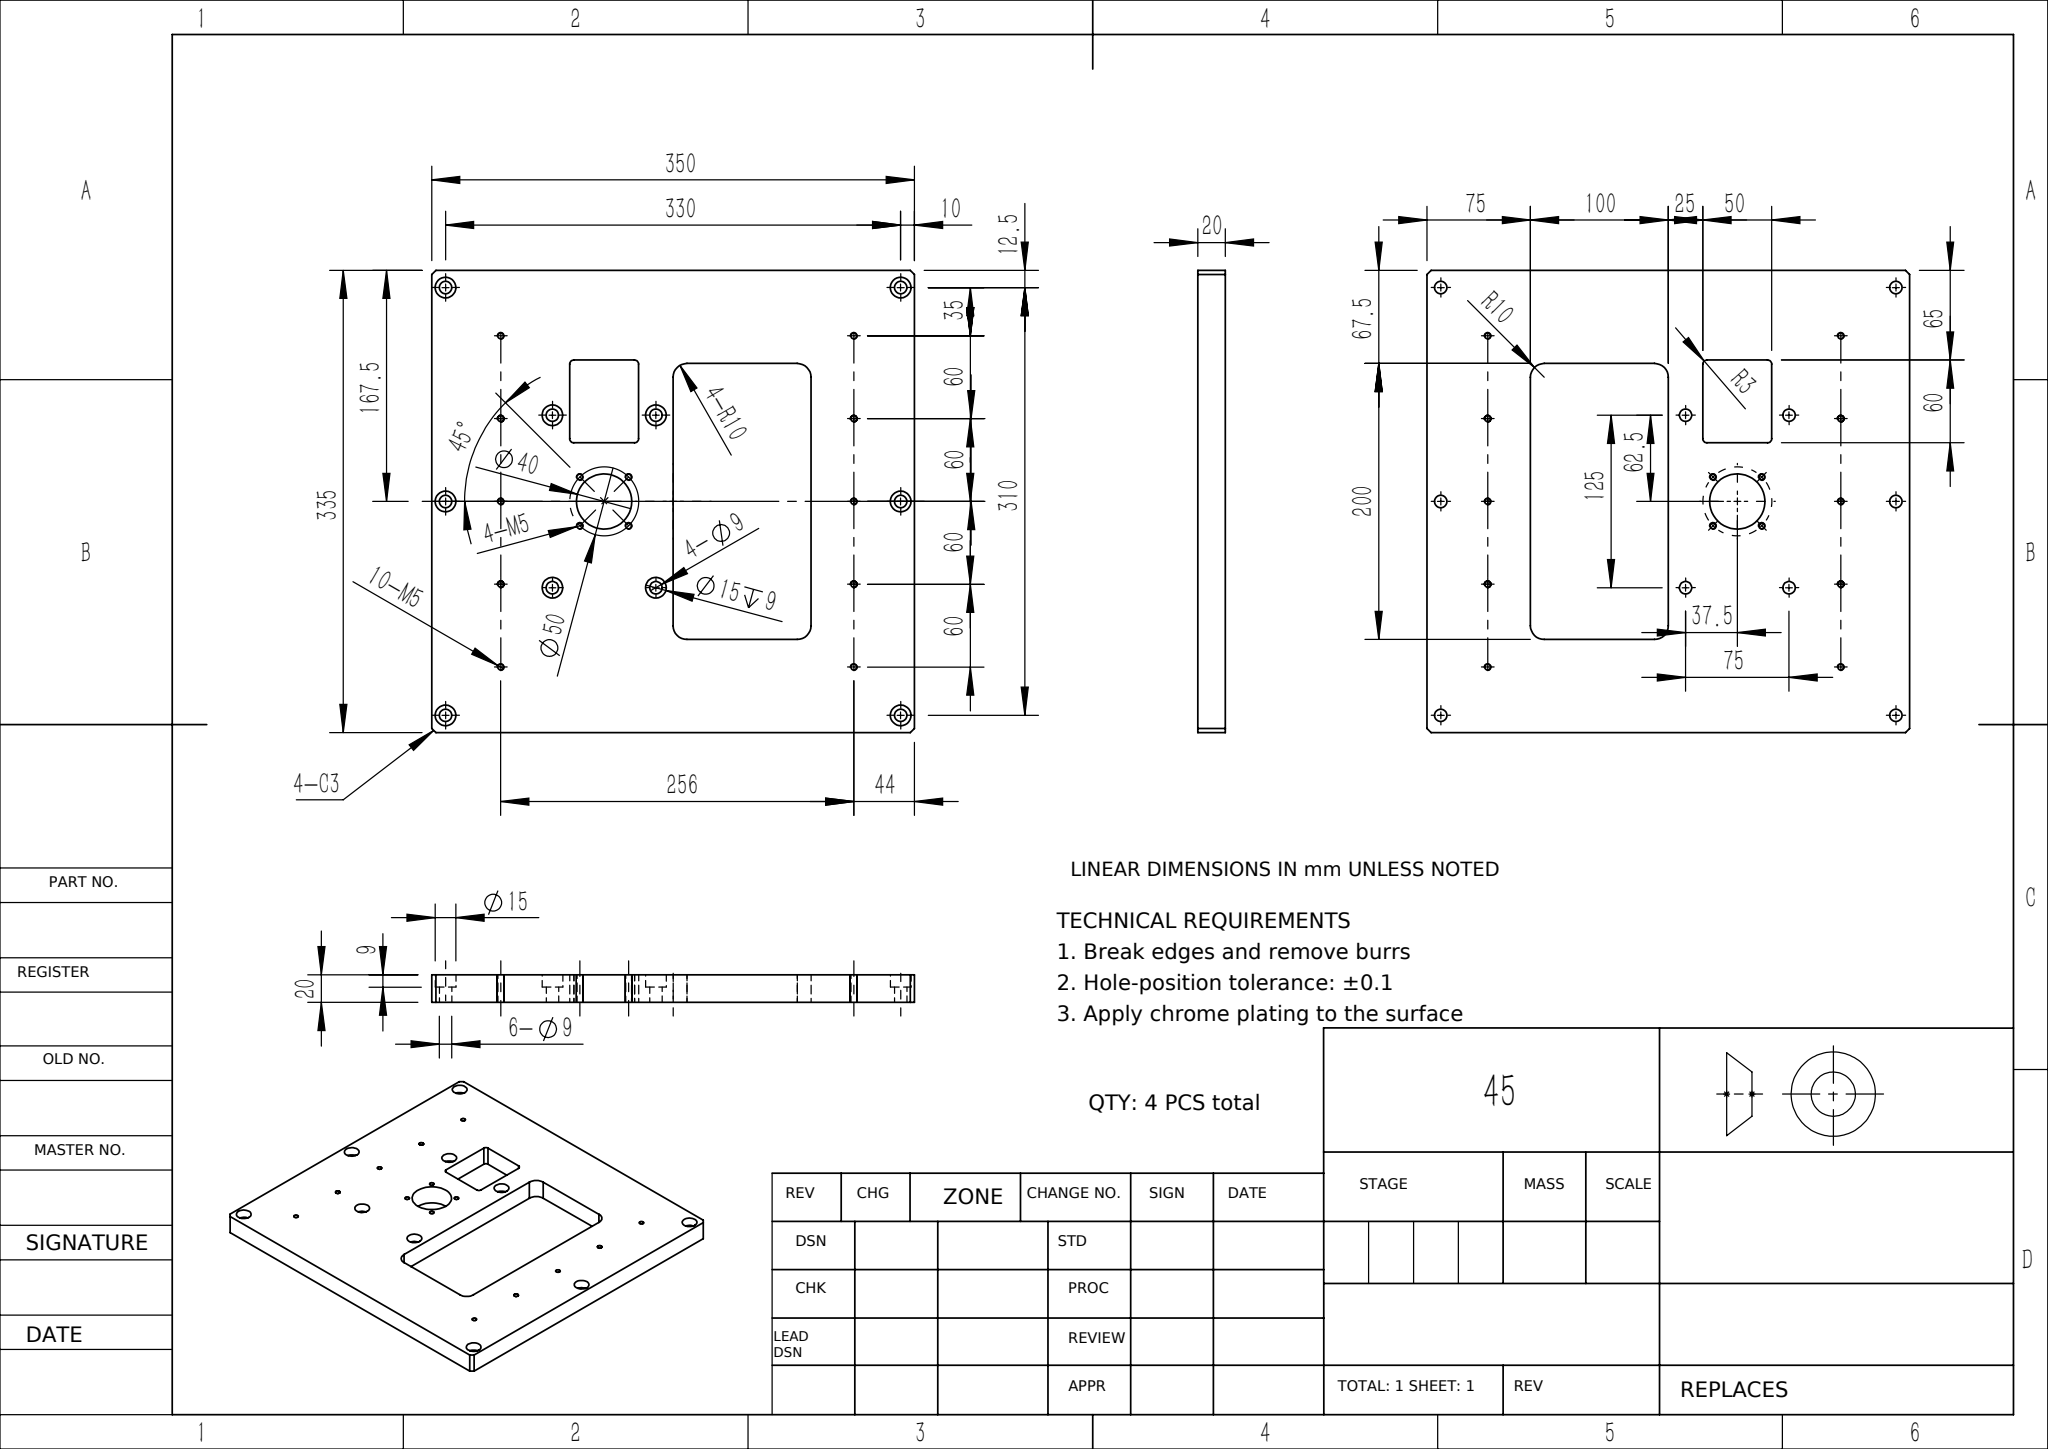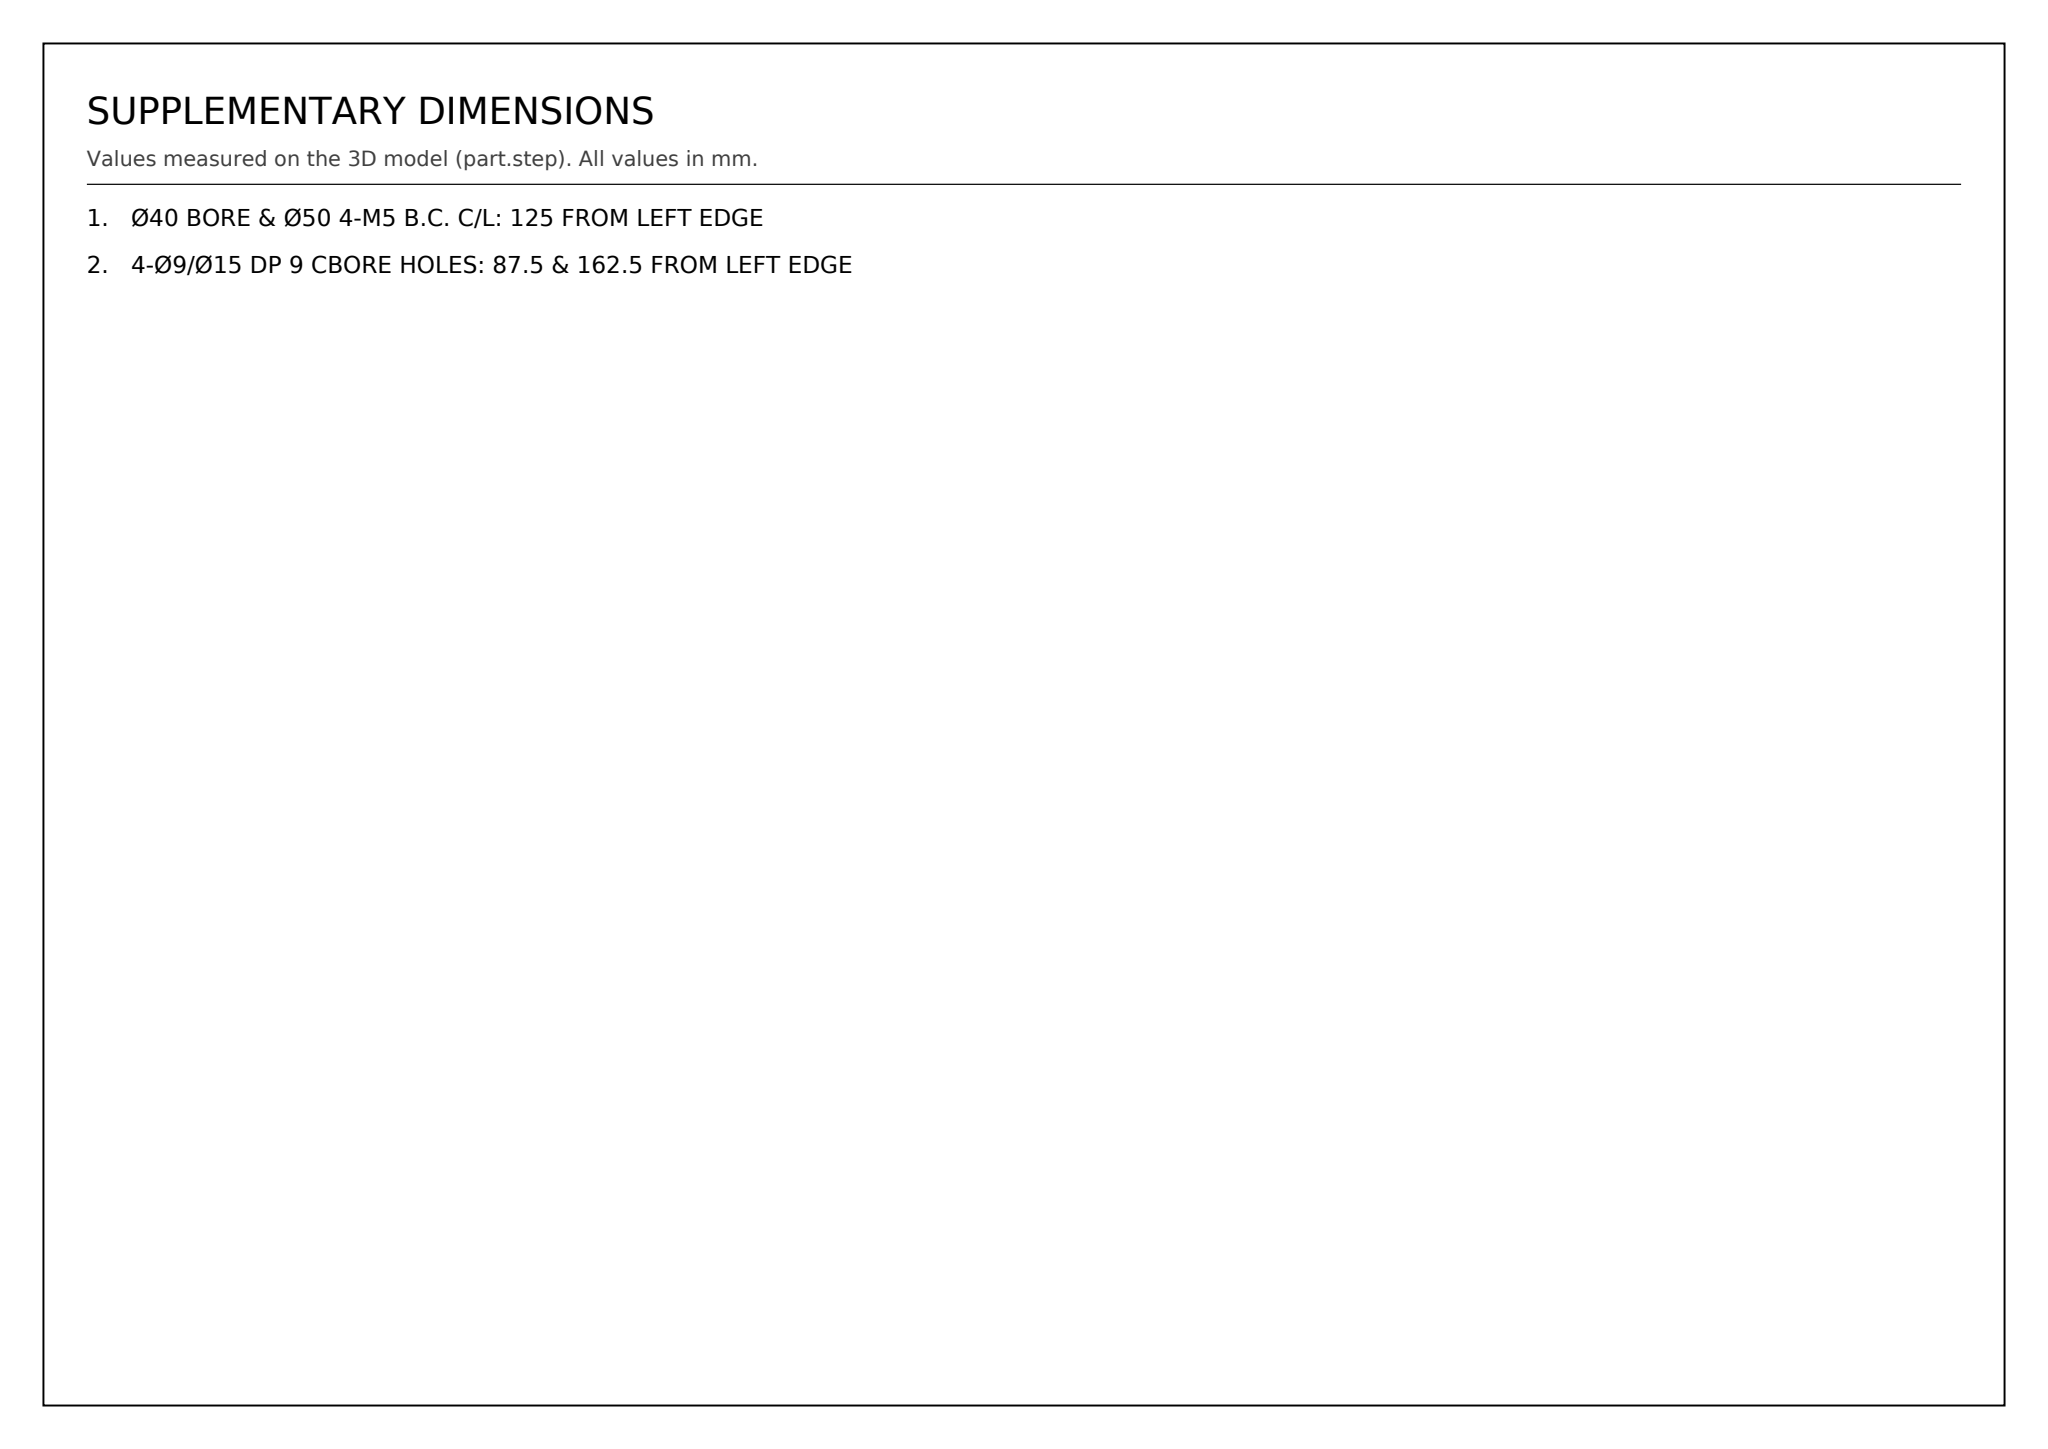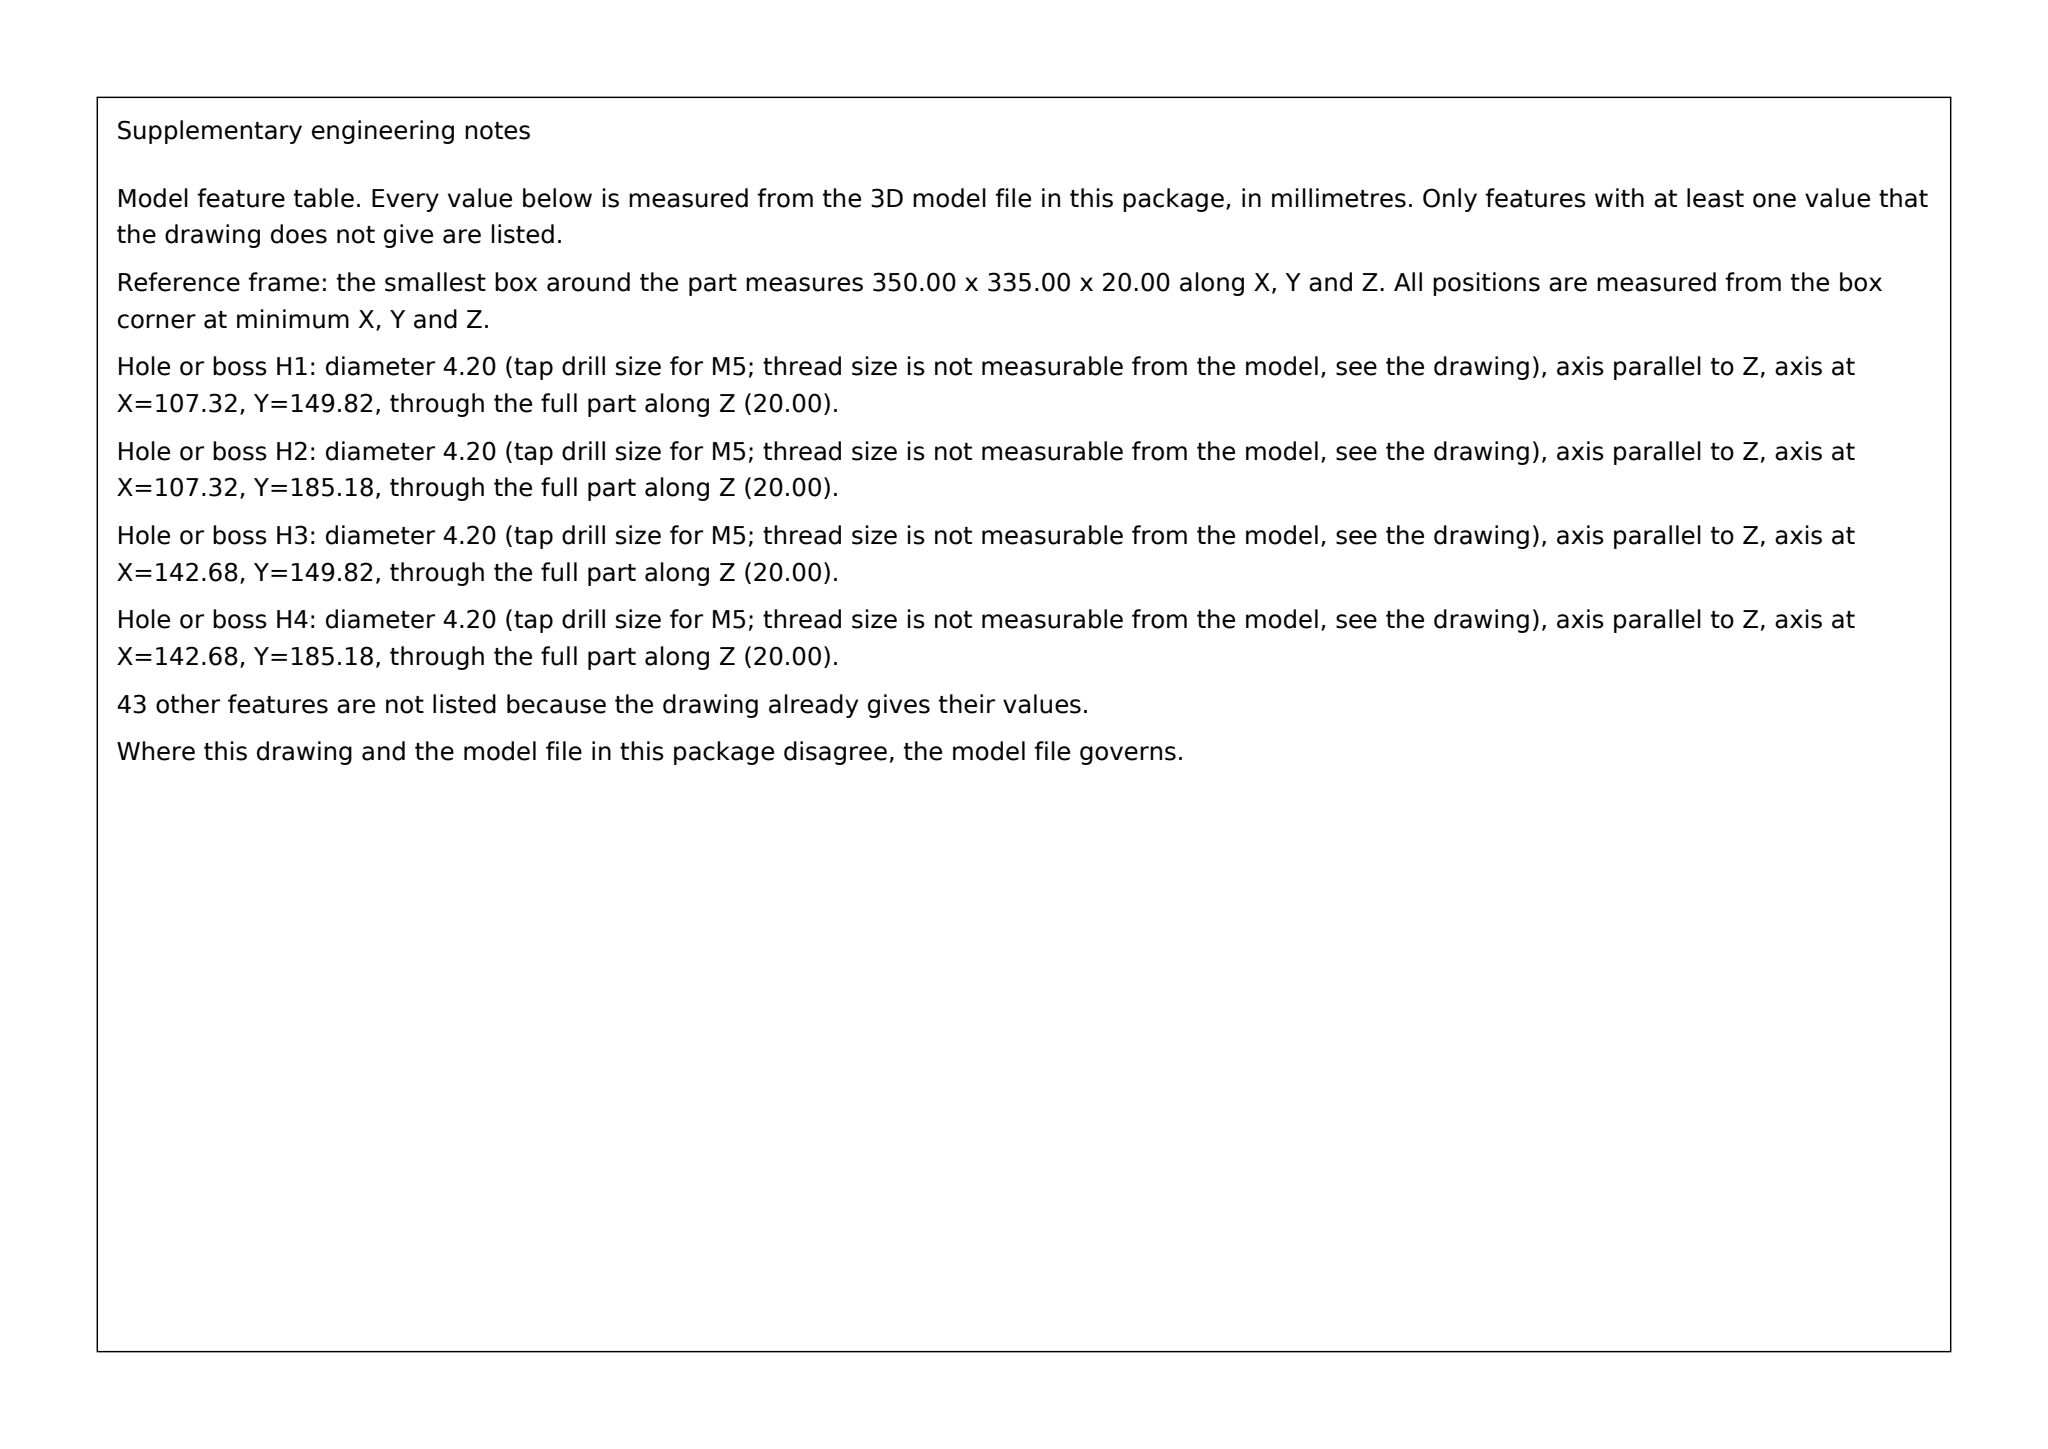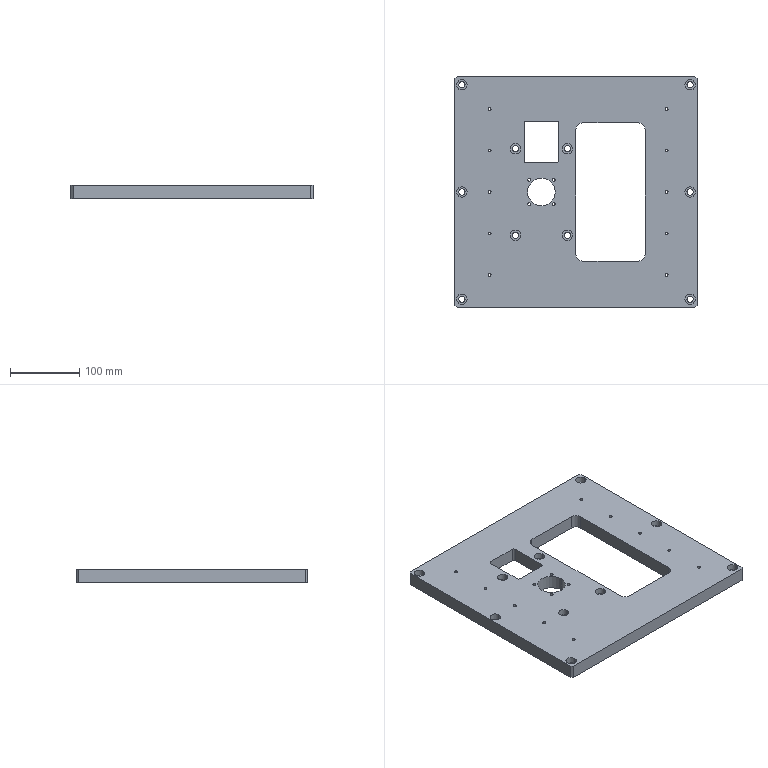Part | SolidWorks | mm | 1 solid | 106 faces | box 350 x 335 x 20 mm | volume 1834597 mm3 | cylinder 78 | plane 28 | commonest cylinder face diameters 4.2 x28 15 x20 9 x20 20 x4 6 x4 40 x2
Drawing notes:
Ø40 BORE & Ø50 4-M5 B.C. C/L: 125 FROM LEFT EDGE | from the solid: Ø40 cyl axis at (125.0, 167.5); M5 Ø4.2 holes at 107.32/142.68 about x=125
4-Ø9/Ø15 DP 9 CBORE HOLES: 87.5 & 162.5 FROM LEFT EDGE | from the solid: Ø9/Ø15 cyls at x=87.5 & 162.5 (y=105 & 230), i.e. 37.5 either side of x=125, 75 apart
build123d program:
from build123d import *

# Parameters (mm, degrees)
SKETCH1_W                                         = 350
SKETCH1_H                                         = 335
BOSS_EXTRUDE1_DEPTH                               = 20
SKETCH2_R                                         = 20
CUT_EXTRUDE1_DEPTH                                = 244.066
M5_TAPPED_HOLE1_D                                 = 4.2
CIRPATTERN1_COUNT                                 = 4
SKETCH5_W                                         = 100
SKETCH5_H                                         = 200
CUT_EXTRUDE2_DEPTH                                = 244.066
FILLET1_R                                         = 10
M5_TAPPED_HOLE2_D                                 = 4.2
LPATTERN1_COUNT                                   = 3
LPATTERN1_PITCH                                   = 60
LPATTERN1_COL_COUNT                               = 3
LPATTERN1_COL_PITCH                               = 60
HOLE_SIZE_ACCORDING_TO_HEX_SOCKET_HEA_D           = 9
HOLE_SIZE_ACCORDING_TO_HEX_SOCKET_HEA_CBORE_D     = 15
HOLE_SIZE_ACCORDING_TO_HEX_SOCKET_HEA_CBORE_DEPTH = 9
CHAMFER1_SIZE                                     = 3
CUT_EXTRUDE3_DEPTH                                = 244.066
HOLE_SIZE_ACCORDING_TO_HEX_SOCKET_2_D             = 9
HOLE_SIZE_ACCORDING_TO_HEX_SOCKET_2_CBORE_D       = 15
HOLE_SIZE_ACCORDING_TO_HEX_SOCKET_2_CBORE_DEPTH   = 9


with BuildPart() as part:
    # Sketch1 → Boss-Extrude1 (new body)
    with BuildSketch(Plane.XY):
        Rectangle(SKETCH1_W, SKETCH1_H)
    extrude(amount=BOSS_EXTRUDE1_DEPTH)

    # Sketch2 → Cut-Extrude1 (cut, through all)
    with BuildSketch(Plane.XY.offset(20)):
        with Locations((-50, 0)):
            Circle(SKETCH2_R)
    extrude(amount=-CUT_EXTRUDE1_DEPTH, mode=Mode.SUBTRACT)

    # M5 Tapped Hole1 (through all)
    with Locations(Plane.XY.offset(20)):
        with Locations((-32.322, 17.678)):
            m5_tapped_hole1 = Hole(M5_TAPPED_HOLE1_D / 2)

    # CirPattern1: M5 Tapped Hole1 ×4 about axis
    cirpattern1_axis = Axis((-50, 0, 0), (0, 0, 1))
    for i in range(1, CIRPATTERN1_COUNT):
        add(m5_tapped_hole1.rotate(cirpattern1_axis, i * 360 / CIRPATTERN1_COUNT), mode=Mode.SUBTRACT)

    # Sketch5 → Cut-Extrude2 (cut, through all)
    with BuildSketch(Plane.XY.offset(20)):
        with Locations((50, 0)):
            Rectangle(SKETCH5_W, SKETCH5_H)
    extrude(amount=-CUT_EXTRUDE2_DEPTH, mode=Mode.SUBTRACT)

    # Fillet1
    fillet1_edges = [part.edges().sort_by_distance(p)[0] for p in [
        (100, 100, 10),
        (100, -100, 10),
        (0, -100, 10),
        (0, 100, 10),
    ]]
    fillet(fillet1_edges, radius=FILLET1_R)

    # M5 Tapped Hole2 (through all)
    with Locations(Plane.XY.offset(20)):
        with Locations((-125, 0), (131, 0)):
            m5_tapped_hole2 = Hole(M5_TAPPED_HOLE2_D / 2)

    # LPattern1: M5 Tapped Hole2 ×3
    with Locations(*[(0, i * LPATTERN1_PITCH, 0) for i in range(1, LPATTERN1_COUNT)]):
        add(m5_tapped_hole2, mode=Mode.SUBTRACT)

    # LPattern1 col: M5 Tapped Hole2 ×3
    with Locations(*[(0, -i * LPATTERN1_COL_PITCH, 0) for i in range(1, LPATTERN1_COL_COUNT)]):
        add(m5_tapped_hole2, mode=Mode.SUBTRACT)

    # Hole Size _ according to_ Hex Socket Hea (through all)
    with Locations(Plane.XY.offset(20)):
        with Locations((165, 155), (-165, 155), (-165, -155), (165, -155), (-165, 0), (165, 0)):
            CounterBoreHole(HOLE_SIZE_ACCORDING_TO_HEX_SOCKET_HEA_D / 2, HOLE_SIZE_ACCORDING_TO_HEX_SOCKET_HEA_CBORE_D / 2, HOLE_SIZE_ACCORDING_TO_HEX_SOCKET_HEA_CBORE_DEPTH)

    # Chamfer1
    chamfer1_edges = [part.edges().sort_by_distance(p)[0] for p in [
        (175, -167.5, 10),
        (-175, -167.5, 10),
        (-175, 167.5, 10),
        (175, 167.5, 10),
    ]]
    chamfer(chamfer1_edges, length=CHAMFER1_SIZE)

    # Sketch10 → Cut-Extrude3 (cut, through all)
    with BuildSketch(Plane.XY.offset(20)):
        with BuildLine():
            Line((-28, 102.5), (-72, 102.5))
            ThreePointArc((-72, 102.5), (-74.121, 101.621), (-75, 99.5))
            Line((-75, 99.5), (-75, 45.5))
            ThreePointArc((-75, 45.5), (-74.121, 43.379), (-72, 42.5))
            Line((-72, 42.5), (-28, 42.5))
            ThreePointArc((-28, 42.5), (-25.879, 43.379), (-25, 45.5))
            Line((-25, 45.5), (-25, 99.5))
            ThreePointArc((-25, 99.5), (-25.879, 101.621), (-28, 102.5))
        make_face()
    extrude(amount=-CUT_EXTRUDE3_DEPTH, mode=Mode.SUBTRACT)

    # Hole Size _ according to_ Hex Socket 2 (through all)
    with Locations(Plane.XY.offset(20)):
        with Locations((-50, 0), (-12.5, -62.5), (-87.5, 62.5), (-87.5, -62.5), (-12.5, 62.5)):
            CounterBoreHole(HOLE_SIZE_ACCORDING_TO_HEX_SOCKET_2_D / 2, HOLE_SIZE_ACCORDING_TO_HEX_SOCKET_2_CBORE_D / 2, HOLE_SIZE_ACCORDING_TO_HEX_SOCKET_2_CBORE_DEPTH)


solid = part.part